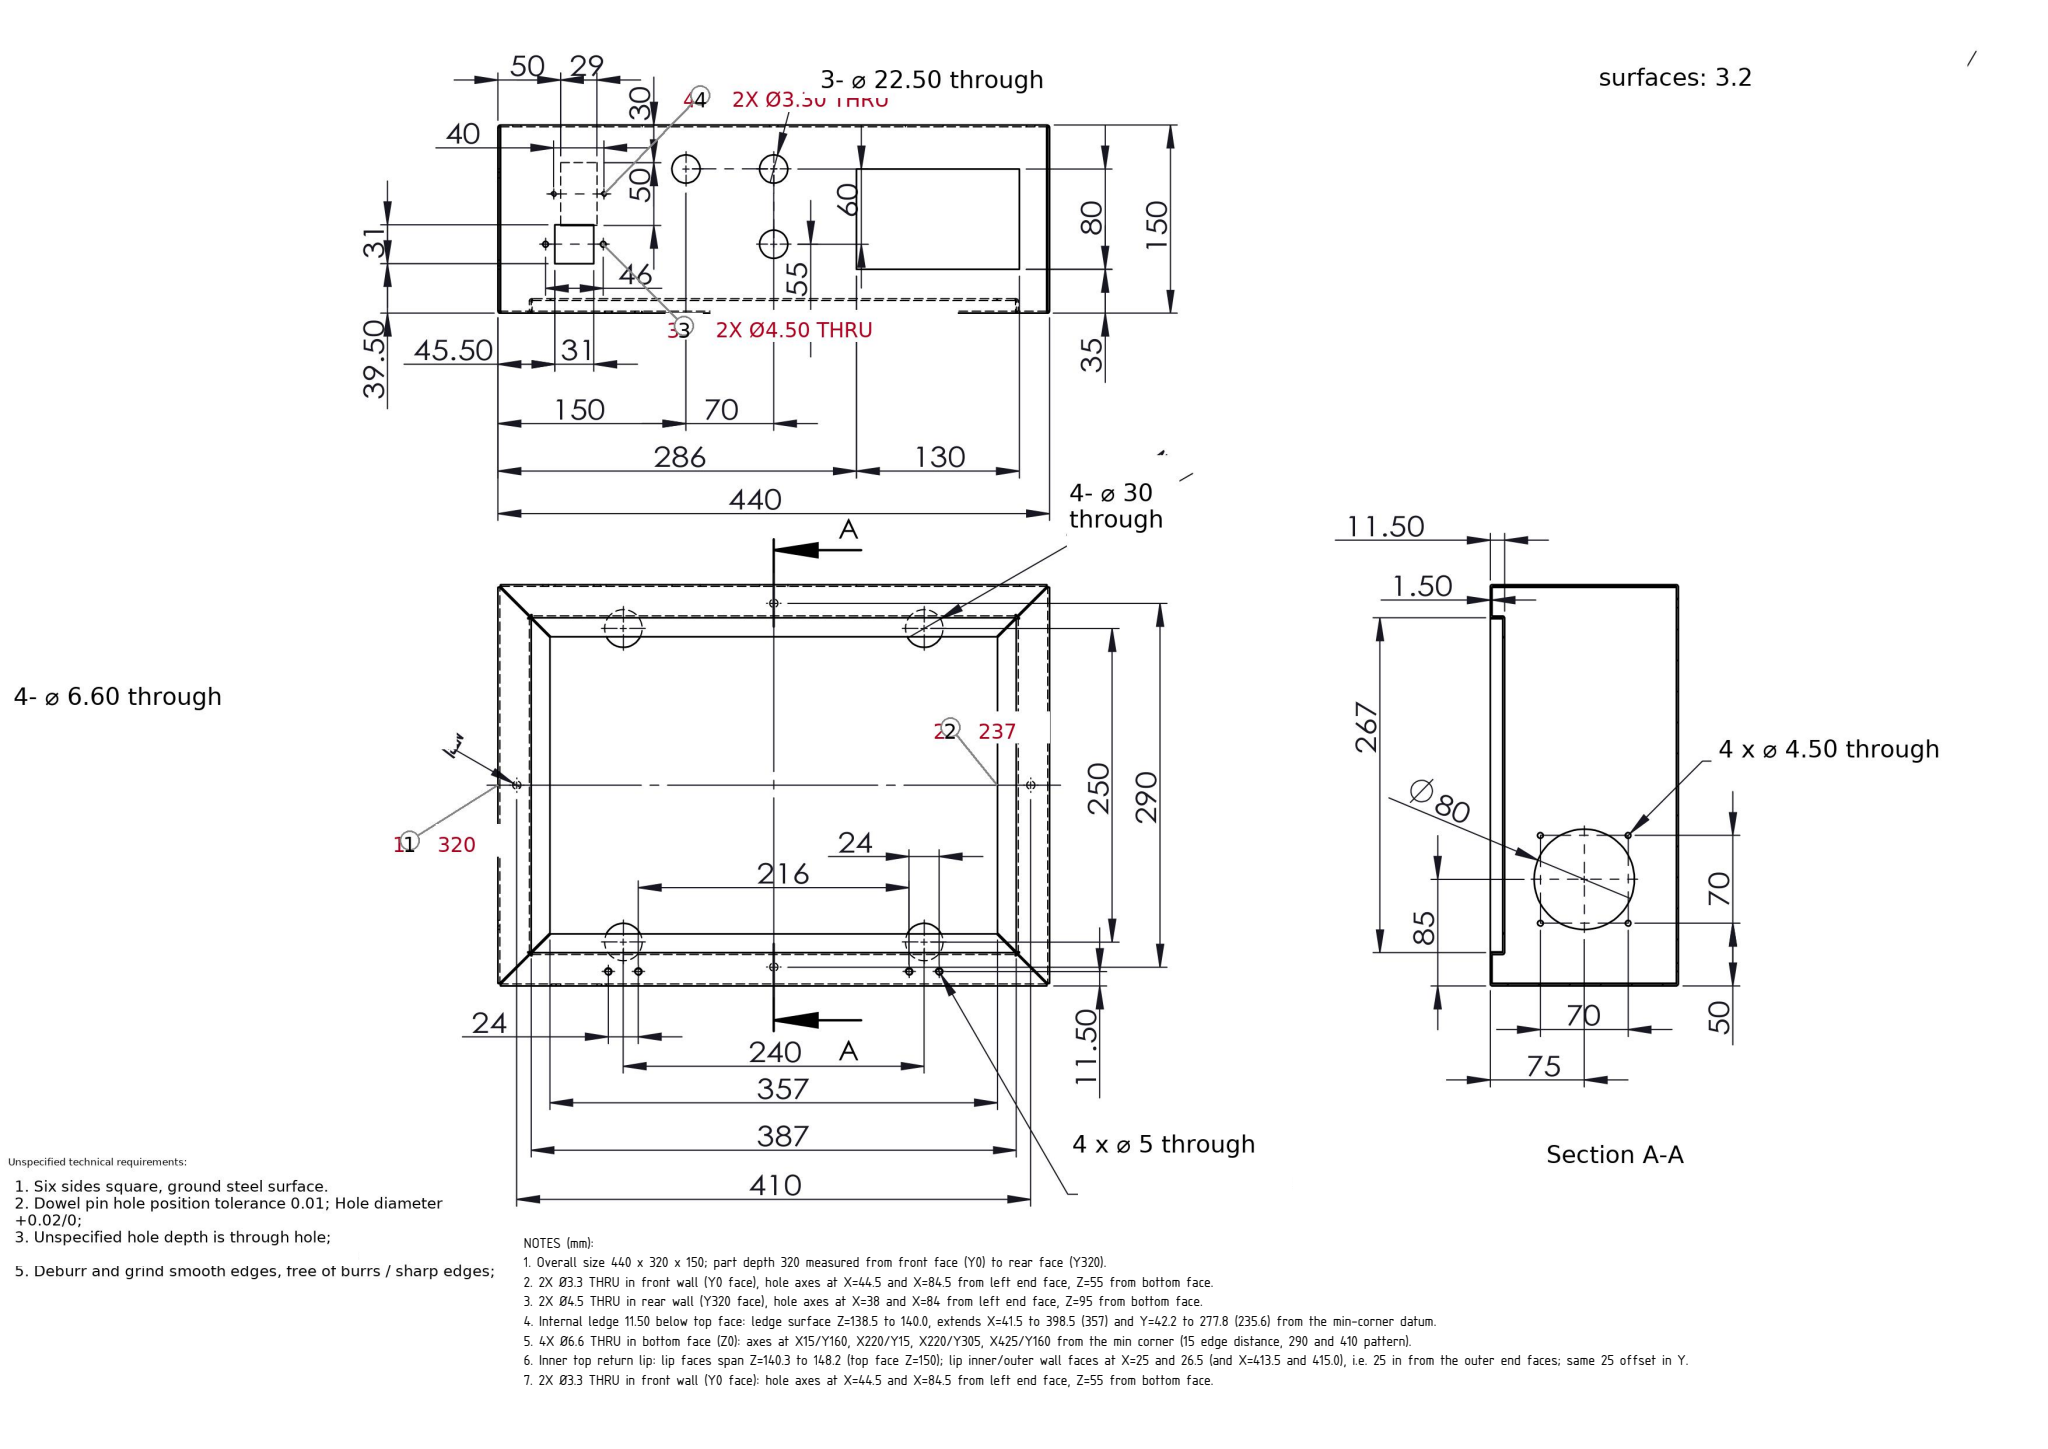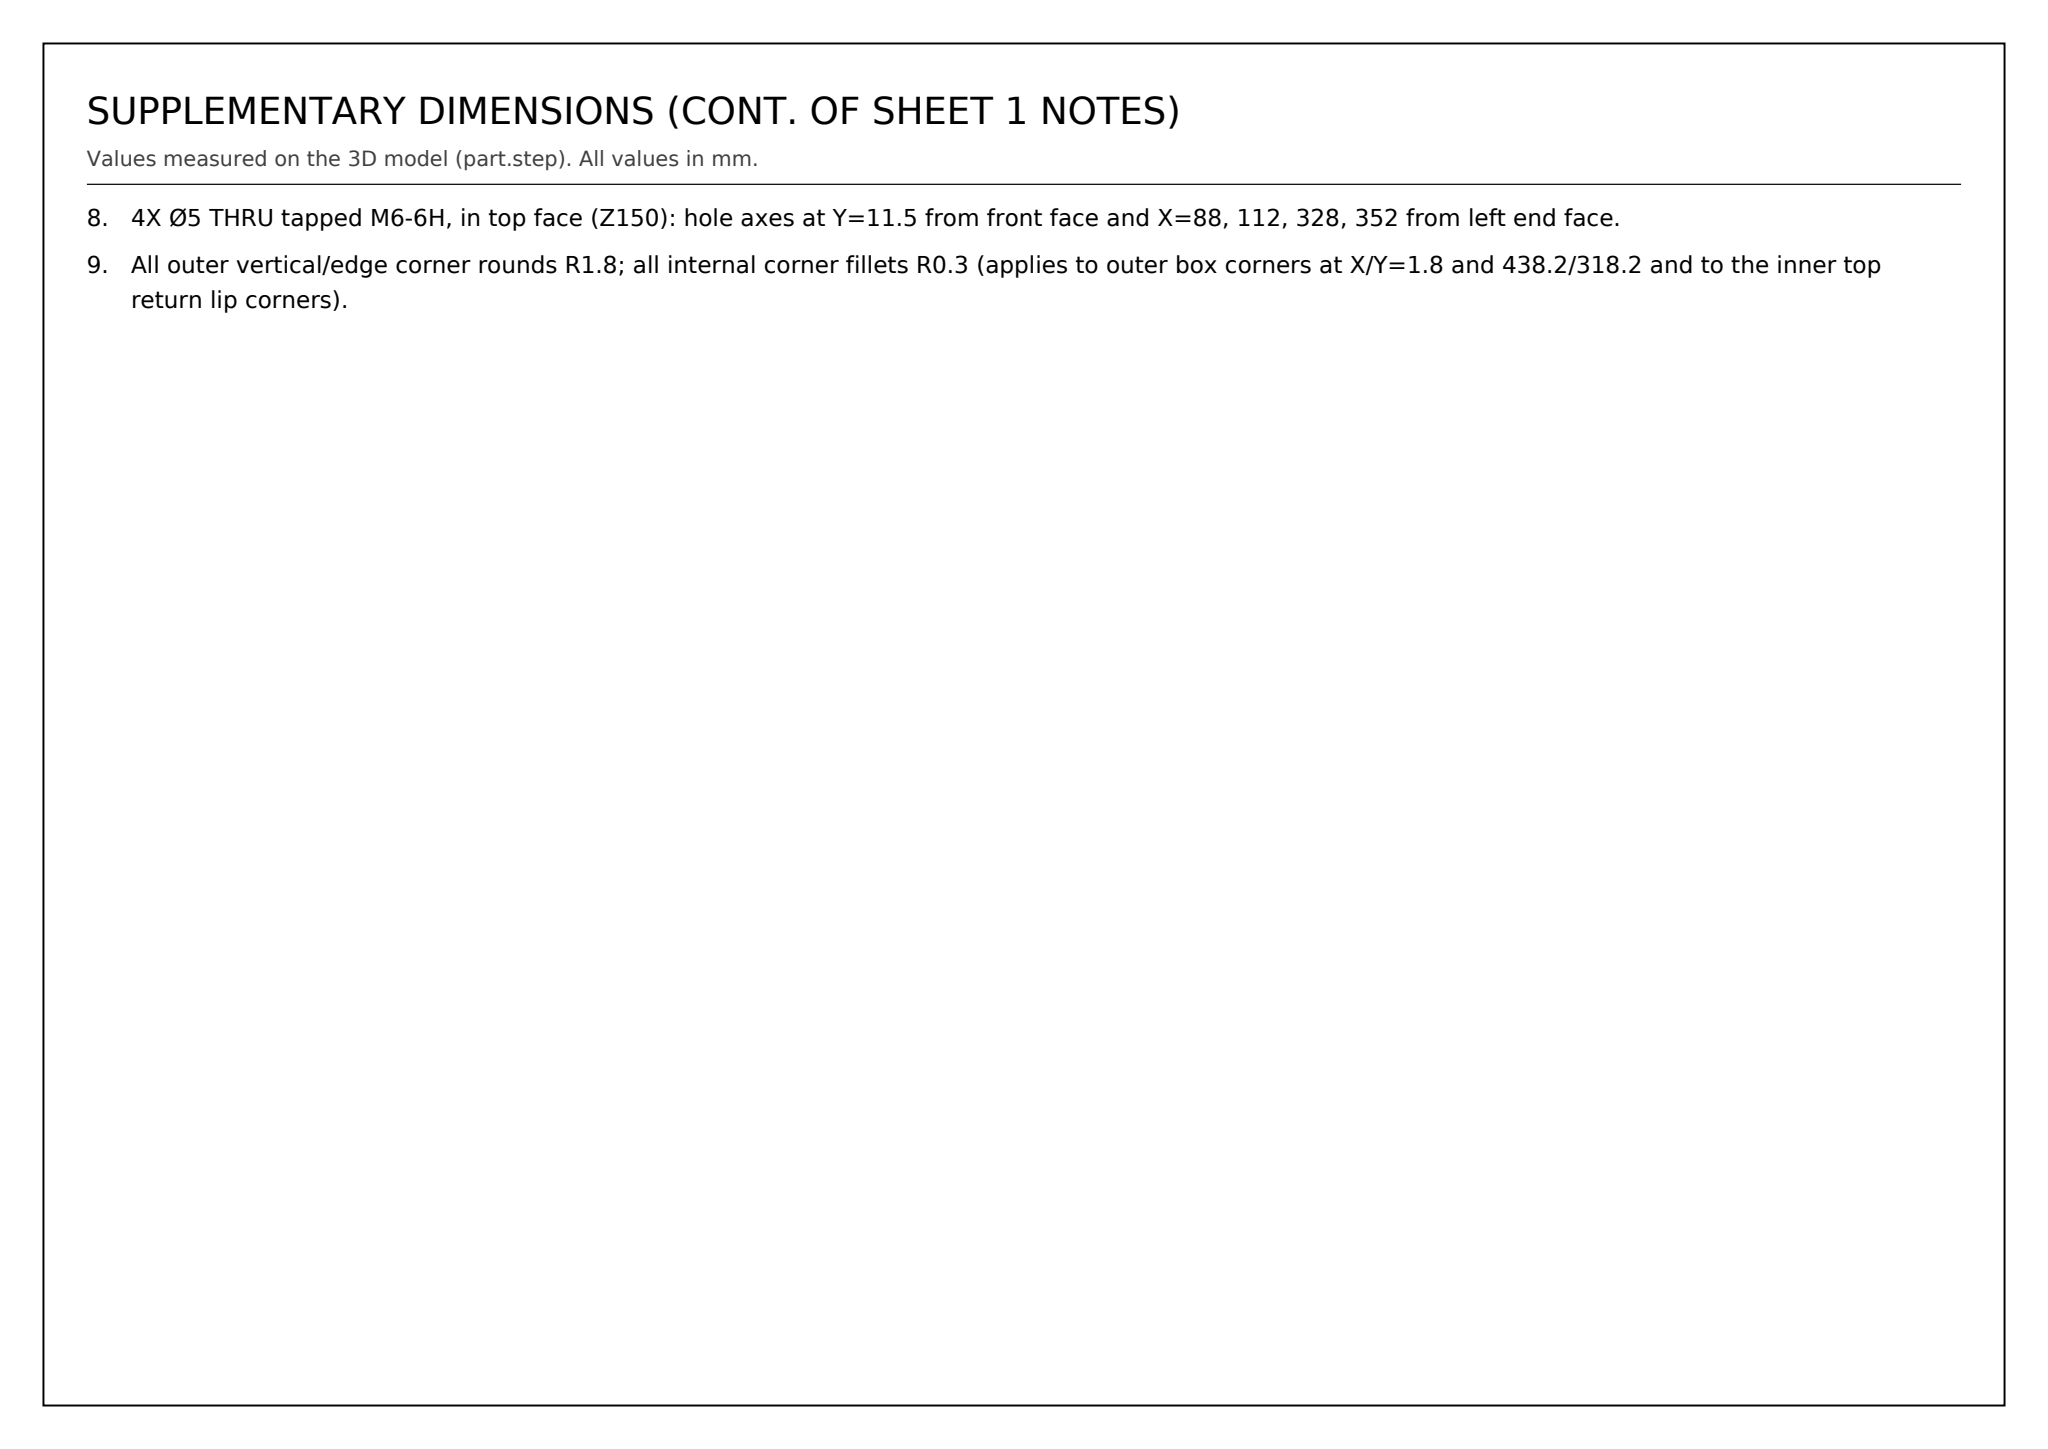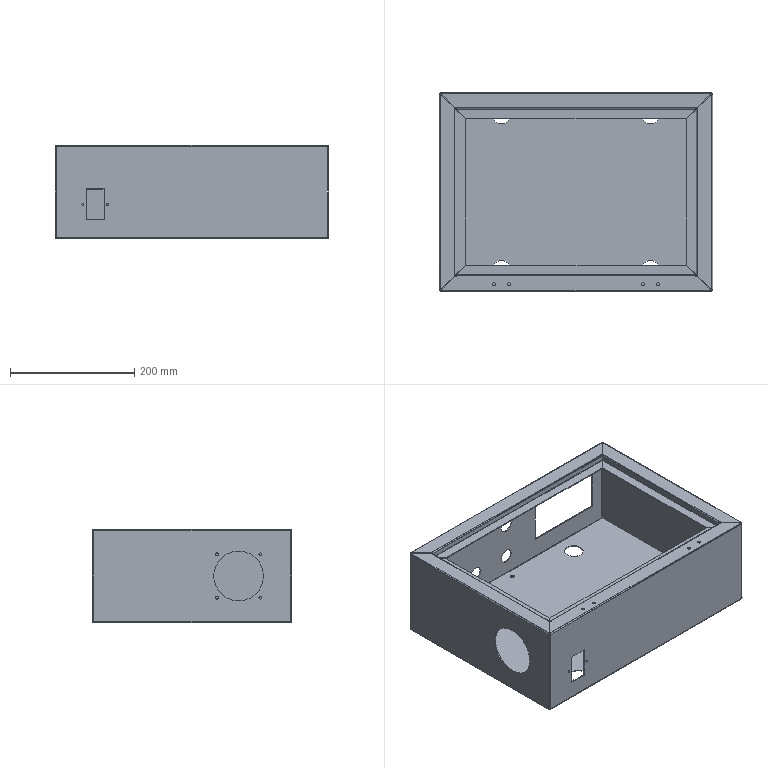Part | SolidWorks | mm | 1 solid | 218 faces | box 440 x 320 x 150 mm | volume 608803 mm3 | plane 114 | cylinder 80 | spline 24 | commonest cylinder face diameters 3.6 x16 0.6 x16 4.5 x12 30 x8 5 x8 6.6 x8 22.5 x6 3.3 x4
Drawing notes:
Overall size 440 x 320 x 150; part depth 320 measured from front face (Y0) to rear face (Y320). | from the solid: bbox_xyz = [440.03, 320.03, 150.03]
2X Ø3.3 THRU in front wall (Y0 face), hole axes at X=44.5 and X=84.5 from left end face, Z=55 from bottom face. | from the solid: cylinders: hole/bore dia 3.3 axis y at [44.5,-,55] and [84.5,-,55], from y0.0 to y1.5
2X Ø4.5 THRU in rear wall (Y320 face), hole axes at X=38 and X=84 from left end face, Z=95 from bottom face. | from the solid: cylinders: hole/bore dia 4.5 axis y at [38.0,-,95.0] and [84.0,-,95.0], from y318.5 to y320.0
Internal ledge 11.50 below top face: ledge surface Z=138.5 to 140.0, extends X=41.5 to 398.5 (357) and Y=42.2 to 277.8 (235.6) from the min-corner datum. | from the solid: axis_planes: x=41.5 and x=398.5, extent y [42.2,277.8], z [138.5,140.0], area 353
4X Ø6.6 THRU in bottom face (Z0): axes at X15/Y160, X220/Y15, X220/Y305, X425/Y160 from the min corner (15 edge distance, 290 and 410 pattern). | from the solid: cylinders: hole/bore dia 6.6 axis z at [15,160], [220,15], [220,305], [425,160], from z0.0 to z1.5
Inner top return lip: lip faces span Z=140.3 to 148.2 (top face Z=150); lip inner/outer wall faces at X=25 and 26.5 (and X=413.5 and 415.0), i.e. 25 in from the outer end faces; same 25 offset in Y. | from the solid: axis_planes x=25.0, x=26.5, x=413.5, x=415.0 with extent z [140.3,148.2]; bbox x 440.03, z 150.03
2X Ø3.3 THRU in front wall (Y0 face): hole axes at X=44.5 and X=84.5 from left end face, Z=55 from bottom face. | from the solid: cylinders: hole/bore dia 3.3, axis y, at [44.5,-,55] and [84.5,-,55], from y=0.0 to 1.5
4X Ø5 THRU tapped M6-6H, in top face (Z150): hole axes at Y=11.5 from front face and X=88, 112, 328, 352 from left end face. | from the solid: cylinders: hole/bore dia 5.0, axis z, at [88,11.5], [112,11.5], [328,11.5], [352,11.5], from z=148.5 to 150.0
All outer vertical/edge corner rounds R1.8; all internal corner fillets R0.3 (applies to outer box corners at X/Y=1.8 and 438.2/318.2 and to the inner top return lip corners). | from the solid: cylinders: convex arc (round/outer radius) dia 3.6 (=R1.8) and concave arc (fillet) dia 0.6 (=R0.3) along x and y edges